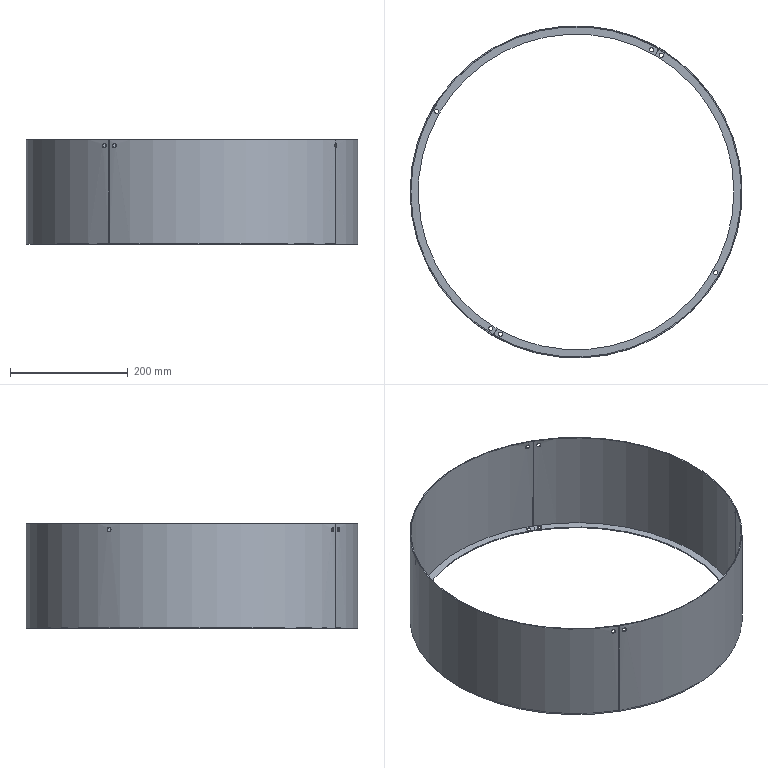Component | SolidWorks | KLHFH026SynchronousBeltCover-1 | 2 solids | 43 faces | volume 500938 mm3 | cylinder 33 | plane 10 | commonest cylinder face diameters 7 x24 535 x3 563 x3 560 x3 | material AISI 304